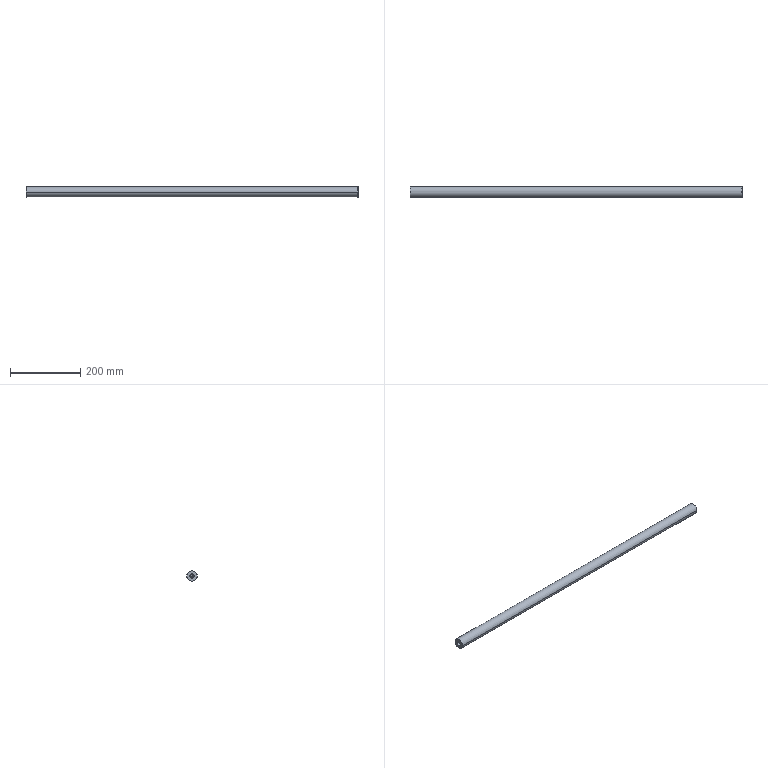Component | SolidWorks | FixedLengthRod-1 | 1 solid | 16 faces | box 944 x 30 x 30 mm | volume 659289 mm3 | cone 8 | cylinder 6 | plane 2 | commonest cylinder face diameters 12 x4 30 x2
build123d program:
from build123d import *

# Parameters (mm, degrees)
SKETCH1_R              = 15
BOSS_EXTRUDE1_DEPTH    = 944
CHAMFER1_SIZE          = 0.5
M14_TAPPED_HOLE1_D     = 12
M14_TAPPED_HOLE1_DEPTH = 34
M14_TAPPED_HOLE1_TIP   = 3.605
M14_TAPPED_HOLE2_D     = 12
M14_TAPPED_HOLE2_DEPTH = 34
M14_TAPPED_HOLE2_TIP   = 3.605


with BuildPart() as part:
    # Sketch1 → Boss-Extrude1 (new body)
    with BuildSketch(Plane.XY):
        Circle(SKETCH1_R)
    extrude(amount=BOSS_EXTRUDE1_DEPTH)

    # Chamfer1
    chamfer1_edges = [part.edges().sort_by_distance(p)[0] for p in [
        (-15, 0, 0),
        (-15, 0, 944),
    ]]
    chamfer(chamfer1_edges, length=CHAMFER1_SIZE)

    # M14 Tapped Hole1
    with Locations(Plane(origin=(0, 0, 0), x_dir=(-1, 0, 0), z_dir=(0, 0, -1))):
        with Locations((0, 0)):
            Hole(M14_TAPPED_HOLE1_D / 2, depth=M14_TAPPED_HOLE1_DEPTH)
            with Locations((0, 0, -(M14_TAPPED_HOLE1_DEPTH + M14_TAPPED_HOLE1_TIP / 2))):  # 118° drill point
                Cone(0, M14_TAPPED_HOLE1_D / 2, M14_TAPPED_HOLE1_TIP, mode=Mode.SUBTRACT)

    # M14 Tapped Hole2
    with Locations(Plane.XY.offset(944)):
        with Locations((0, 0)):
            Hole(M14_TAPPED_HOLE2_D / 2, depth=M14_TAPPED_HOLE2_DEPTH)
            with Locations((0, 0, -(M14_TAPPED_HOLE2_DEPTH + M14_TAPPED_HOLE2_TIP / 2))):  # 118° drill point
                Cone(0, M14_TAPPED_HOLE2_D / 2, M14_TAPPED_HOLE2_TIP, mode=Mode.SUBTRACT)


solid = part.part

# Placed as in the assembly
solid = solid.moved(Location((-625.02, -279.181, 155), (0, 90, 0)))
STEP:
#1=CARTESIAN_POINT('',(-23.269,-11.228,6.102));
#2=VERTEX_POINT('',#1);
#3=CARTESIAN_POINT('',(-23.269,-10.755,6.102));
#4=VERTEX_POINT('',#3);
#5=CARTESIAN_POINT('',(-23.269,-10.991,6.102));
#6=DIRECTION('',(-1.,0.,0.));
#7=DIRECTION('',(0.,1.,0.));
#8=AXIS2_PLACEMENT_3D('',#5,#6,#7);
#9=CIRCLE('',#8,0.2362);
#10=EDGE_CURVE('',#2,#4,#9,.T.);
#11=ORIENTED_EDGE('',*,*,#10,.F.);
#12=CARTESIAN_POINT('',(-24.607,-11.228,6.102));
#13=VERTEX_POINT('',#12);
#14=CARTESIAN_POINT('',(-24.607,-11.228,6.102));
#15=DIRECTION('',(-1.,0.,0.));
#16=VECTOR('',#15,39.37);
#17=LINE('',#14,#16);
#18=EDGE_CURVE('',#2,#13,#17,.T.);
#19=ORIENTED_EDGE('',*,*,#18,.T.);
#20=CARTESIAN_POINT('',(-24.607,-10.755,6.102));
#21=VERTEX_POINT('',#20);
#22=CARTESIAN_POINT('',(-24.607,-10.991,6.102));
#23=DIRECTION('',(-1.,0.,0.));
#24=DIRECTION('',(0.,1.,0.));
#25=AXIS2_PLACEMENT_3D('',#22,#23,#24);
#26=CIRCLE('',#25,0.2362);
#27=EDGE_CURVE('',#13,#21,#26,.T.);
#28=ORIENTED_EDGE('',*,*,#27,.T.);
#29=CARTESIAN_POINT('',(-24.607,-10.755,6.102));
#30=DIRECTION('',(-1.,0.,0.));
#31=VECTOR('',#30,39.37);
#32=LINE('',#29,#31);
#33=EDGE_CURVE('',#4,#21,#32,.T.);
#34=ORIENTED_EDGE('',*,*,#33,.F.);
#35=EDGE_LOOP('',(#11,#19,#28,#34));
#36=FACE_OUTER_BOUND('',#35,.T.);
#37=CARTESIAN_POINT('',(-24.607,-10.991,6.102));
#38=DIRECTION('',(-1.,0.,0.));
#39=DIRECTION('',(0.,1.,0.));
#40=AXIS2_PLACEMENT_3D('',#37,#38,#39);
#41=CYLINDRICAL_SURFACE('',#40,0.2362);
#42=ADVANCED_FACE('',(#36),#41,.F.);
#43=CARTESIAN_POINT('',(-23.127,-10.991,6.102));
#44=VERTEX_POINT('',#43);
#45=CARTESIAN_POINT('',(-23.269,-10.755,6.102));
#46=DIRECTION('',(-0.515,0.8572,0.));
#47=VECTOR('',#46,39.37);
#48=LINE('',#45,#47);
#49=EDGE_CURVE('',#44,#4,#48,.T.);
#50=ORIENTED_EDGE('',*,*,#49,.F.);
#51=CARTESIAN_POINT('',(-23.269,-11.228,6.102));
#52=DIRECTION('',(-0.515,-0.8572,-0.));
#53=VECTOR('',#52,39.37);
#54=LINE('',#51,#53);
#55=EDGE_CURVE('',#44,#2,#54,.T.);
#56=ORIENTED_EDGE('',*,*,#55,.T.);
#57=ORIENTED_EDGE('',*,*,#10,.T.);
#58=EDGE_LOOP('',(#50,#56,#57));
#59=FACE_OUTER_BOUND('',#58,.T.);
#60=CARTESIAN_POINT('',(-23.269,-10.991,6.102));
#61=DIRECTION('',(-1.,0.,0.));
#62=DIRECTION('',(0.,1.,0.));
#63=AXIS2_PLACEMENT_3D('',#60,#61,#62);
#64=CONICAL_SURFACE('',#63,0.2362,1.03);
#65=ADVANCED_FACE('',(#59),#64,.F.);
#66=CARTESIAN_POINT('',(11.22,-10.755,6.102));
#67=VERTEX_POINT('',#66);
#68=CARTESIAN_POINT('',(11.22,-11.228,6.102));
#69=VERTEX_POINT('',#68);
#70=CARTESIAN_POINT('',(11.22,-10.991,6.102));
#71=DIRECTION('',(1.,0.,0.));
#72=DIRECTION('',(0.,-1.,0.));
#73=AXIS2_PLACEMENT_3D('',#70,#71,#72);
#74=CIRCLE('',#73,0.2362);
#75=EDGE_CURVE('',#67,#69,#74,.T.);
#76=ORIENTED_EDGE('',*,*,#75,.F.);
#77=CARTESIAN_POINT('',(12.558,-10.755,6.102));
#78=VERTEX_POINT('',#77);
#79=CARTESIAN_POINT('',(12.558,-10.755,6.102));
#80=DIRECTION('',(1.,0.,0.));
#81=VECTOR('',#80,39.37);
#82=LINE('',#79,#81);
#83=EDGE_CURVE('',#67,#78,#82,.T.);
#84=ORIENTED_EDGE('',*,*,#83,.T.);
#85=CARTESIAN_POINT('',(12.558,-11.228,6.102));
#86=VERTEX_POINT('',#85);
#87=CARTESIAN_POINT('',(12.558,-10.991,6.102));
#88=DIRECTION('',(1.,0.,0.));
#89=DIRECTION('',(0.,-1.,0.));
#90=AXIS2_PLACEMENT_3D('',#87,#88,#89);
#91=CIRCLE('',#90,0.2362);
#92=EDGE_CURVE('',#78,#86,#91,.T.);
#93=ORIENTED_EDGE('',*,*,#92,.T.);
#94=CARTESIAN_POINT('',(12.558,-11.228,6.102));
#95=DIRECTION('',(1.,0.,0.));
#96=VECTOR('',#95,39.37);
#97=LINE('',#94,#96);
#98=EDGE_CURVE('',#69,#86,#97,.T.);
#99=ORIENTED_EDGE('',*,*,#98,.F.);
#100=EDGE_LOOP('',(#76,#84,#93,#99));
#101=FACE_OUTER_BOUND('',#100,.T.);
#102=CARTESIAN_POINT('',(12.558,-10.991,6.102));
#103=DIRECTION('',(1.,0.,0.));
#104=DIRECTION('',(0.,-1.,0.));
#105=AXIS2_PLACEMENT_3D('',#102,#103,#104);
#106=CYLINDRICAL_SURFACE('',#105,0.2362);
#107=ADVANCED_FACE('',(#101),#106,.F.);
#108=CARTESIAN_POINT('',(11.078,-10.991,6.102));
#109=VERTEX_POINT('',#108);
#110=CARTESIAN_POINT('',(11.22,-11.228,6.102));
#111=DIRECTION('',(0.515,-0.8572,-0.));
#112=VECTOR('',#111,39.37);
#113=LINE('',#110,#112);
#114=EDGE_CURVE('',#109,#69,#113,.T.);
#115=ORIENTED_EDGE('',*,*,#114,.F.);
#116=CARTESIAN_POINT('',(11.22,-10.755,6.102));
#117=DIRECTION('',(0.515,0.8572,0.));
#118=VECTOR('',#117,39.37);
#119=LINE('',#116,#118);
#120=EDGE_CURVE('',#109,#67,#119,.T.);
#121=ORIENTED_EDGE('',*,*,#120,.T.);
#122=ORIENTED_EDGE('',*,*,#75,.T.);
#123=EDGE_LOOP('',(#115,#121,#122));
#124=FACE_OUTER_BOUND('',#123,.T.);
#125=CARTESIAN_POINT('',(11.22,-10.991,6.102));
#126=DIRECTION('',(1.,0.,0.));
#127=DIRECTION('',(0.,-1.,0.));
#128=AXIS2_PLACEMENT_3D('',#125,#126,#127);
#129=CONICAL_SURFACE('',#128,0.2362,1.03);
#130=ADVANCED_FACE('',(#124),#129,.F.);
#131=CARTESIAN_POINT('',(-24.607,-10.421,6.102));
#132=VERTEX_POINT('',#131);
#133=CARTESIAN_POINT('',(-24.607,-11.562,6.102));
#134=VERTEX_POINT('',#133);
#135=CARTESIAN_POINT('',(-24.607,-10.991,6.102));
#136=DIRECTION('',(-1.,0.,0.));
#137=DIRECTION('',(0.,1.,0.));
#138=AXIS2_PLACEMENT_3D('',#135,#136,#137);
#139=CIRCLE('',#138,0.5709);
#140=EDGE_CURVE('',#132,#134,#139,.T.);
#141=ORIENTED_EDGE('',*,*,#140,.F.);
#142=CARTESIAN_POINT('',(-24.587,-10.401,6.102));
#143=VERTEX_POINT('',#142);
#144=CARTESIAN_POINT('',(-24.607,-10.421,6.102));
#145=DIRECTION('',(0.7071,0.7071,0.));
#146=VECTOR('',#145,39.37);
#147=LINE('',#144,#146);
#148=EDGE_CURVE('',#132,#143,#147,.T.);
#149=ORIENTED_EDGE('',*,*,#148,.T.);
#150=CARTESIAN_POINT('',(-24.587,-11.582,6.102));
#151=VERTEX_POINT('',#150);
#152=CARTESIAN_POINT('',(-24.587,-10.991,6.102));
#153=DIRECTION('',(1.,0.,0.));
#154=DIRECTION('',(0.,1.,0.));
#155=AXIS2_PLACEMENT_3D('',#152,#153,#154);
#156=CIRCLE('',#155,0.5906);
#157=EDGE_CURVE('',#151,#143,#156,.T.);
#158=ORIENTED_EDGE('',*,*,#157,.F.);
#159=CARTESIAN_POINT('',(-24.607,-11.562,6.102));
#160=DIRECTION('',(0.7071,-0.7071,-0.));
#161=VECTOR('',#160,39.37);
#162=LINE('',#159,#161);
#163=EDGE_CURVE('',#134,#151,#162,.T.);
#164=ORIENTED_EDGE('',*,*,#163,.F.);
#165=EDGE_LOOP('',(#141,#149,#158,#164));
#166=FACE_OUTER_BOUND('',#165,.T.);
#167=CARTESIAN_POINT('',(-24.607,-10.991,6.102));
#168=DIRECTION('',(1.,0.,0.));
#169=DIRECTION('',(0.,-1.,-0.));
#170=AXIS2_PLACEMENT_3D('',#167,#168,#169);
#171=CONICAL_SURFACE('',#170,0.5709,0.7854);
#172=ADVANCED_FACE('',(#166),#171,.T.);
#173=CARTESIAN_POINT('',(12.558,-11.562,6.102));
#174=VERTEX_POINT('',#173);
#175=CARTESIAN_POINT('',(12.558,-10.421,6.102));
#176=VERTEX_POINT('',#175);
#177=CARTESIAN_POINT('',(12.558,-10.991,6.102));
#178=DIRECTION('',(1.,0.,0.));
#179=DIRECTION('',(0.,1.,0.));
#180=AXIS2_PLACEMENT_3D('',#177,#178,#179);
#181=CIRCLE('',#180,0.5709);
#182=EDGE_CURVE('',#174,#176,#181,.T.);
#183=ORIENTED_EDGE('',*,*,#182,.F.);
#184=CARTESIAN_POINT('',(12.539,-11.582,6.102));
#185=VERTEX_POINT('',#184);
#186=CARTESIAN_POINT('',(12.539,-11.582,6.102));
#187=DIRECTION('',(-0.7071,-0.7071,-0.));
#188=VECTOR('',#187,39.37);
#189=LINE('',#186,#188);
#190=EDGE_CURVE('',#174,#185,#189,.T.);
#191=ORIENTED_EDGE('',*,*,#190,.T.);
#192=CARTESIAN_POINT('',(12.539,-10.401,6.102));
#193=VERTEX_POINT('',#192);
#194=CARTESIAN_POINT('',(12.539,-10.991,6.102));
#195=DIRECTION('',(-1.,0.,0.));
#196=DIRECTION('',(0.,1.,0.));
#197=AXIS2_PLACEMENT_3D('',#194,#195,#196);
#198=CIRCLE('',#197,0.5906);
#199=EDGE_CURVE('',#193,#185,#198,.T.);
#200=ORIENTED_EDGE('',*,*,#199,.F.);
#201=CARTESIAN_POINT('',(12.539,-10.401,6.102));
#202=DIRECTION('',(-0.7071,0.7071,0.));
#203=VECTOR('',#202,39.37);
#204=LINE('',#201,#203);
#205=EDGE_CURVE('',#176,#193,#204,.T.);
#206=ORIENTED_EDGE('',*,*,#205,.F.);
#207=EDGE_LOOP('',(#183,#191,#200,#206));
#208=FACE_OUTER_BOUND('',#207,.T.);
#209=CARTESIAN_POINT('',(12.539,-10.991,6.102));
#210=DIRECTION('',(-1.,0.,0.));
#211=DIRECTION('',(0.,1.,0.));
#212=AXIS2_PLACEMENT_3D('',#209,#210,#211);
#213=CONICAL_SURFACE('',#212,0.5906,0.7854);
#214=ADVANCED_FACE('',(#208),#213,.T.);
#215=ORIENTED_EDGE('',*,*,#157,.T.);
#216=CARTESIAN_POINT('',(-24.607,-10.401,6.102));
#217=DIRECTION('',(1.,0.,0.));
#218=VECTOR('',#217,39.37);
#219=LINE('',#216,#218);
#220=EDGE_CURVE('',#143,#193,#219,.T.);
#221=ORIENTED_EDGE('',*,*,#220,.T.);
#222=ORIENTED_EDGE('',*,*,#199,.T.);
#223=CARTESIAN_POINT('',(-24.607,-11.582,6.102));
#224=DIRECTION('',(1.,0.,0.));
#225=VECTOR('',#224,39.37);
#226=LINE('',#223,#225);
#227=EDGE_CURVE('',#151,#185,#226,.T.);
#228=ORIENTED_EDGE('',*,*,#227,.F.);
#229=EDGE_LOOP('',(#215,#221,#222,#228));
#230=FACE_OUTER_BOUND('',#229,.T.);
#231=CARTESIAN_POINT('',(-24.607,-10.991,6.102));
#232=DIRECTION('',(1.,0.,0.));
#233=DIRECTION('',(0.,-1.,-0.));
#234=AXIS2_PLACEMENT_3D('',#231,#232,#233);
#235=CYLINDRICAL_SURFACE('',#234,0.5906);
#236=ADVANCED_FACE('',(#230),#235,.T.);
#237=ORIENTED_EDGE('',*,*,#220,.F.);
#238=CARTESIAN_POINT('',(-24.587,-10.991,6.102));
#239=DIRECTION('',(1.,0.,0.));
#240=DIRECTION('',(0.,1.,0.));
#241=AXIS2_PLACEMENT_3D('',#238,#239,#240);
#242=CIRCLE('',#241,0.5906);
#243=EDGE_CURVE('',#143,#151,#242,.T.);
#244=ORIENTED_EDGE('',*,*,#243,.T.);
#245=ORIENTED_EDGE('',*,*,#227,.T.);
#246=CARTESIAN_POINT('',(12.539,-10.991,6.102));
#247=DIRECTION('',(-1.,0.,0.));
#248=DIRECTION('',(0.,1.,0.));
#249=AXIS2_PLACEMENT_3D('',#246,#247,#248);
#250=CIRCLE('',#249,0.5906);
#251=EDGE_CURVE('',#185,#193,#250,.T.);
#252=ORIENTED_EDGE('',*,*,#251,.T.);
#253=EDGE_LOOP('',(#237,#244,#245,#252));
#254=FACE_OUTER_BOUND('',#253,.T.);
#255=CARTESIAN_POINT('',(-24.607,-10.991,6.102));
#256=DIRECTION('',(1.,0.,0.));
#257=DIRECTION('',(0.,-1.,-0.));
#258=AXIS2_PLACEMENT_3D('',#255,#256,#257);
#259=CYLINDRICAL_SURFACE('',#258,0.5906);
#260=ADVANCED_FACE('',(#254),#259,.T.);
#261=CARTESIAN_POINT('',(-24.607,-10.991,6.102));
#262=DIRECTION('',(-1.,0.,0.));
#263=DIRECTION('',(0.,1.,0.));
#264=AXIS2_PLACEMENT_3D('',#261,#262,#263);
#265=CIRCLE('',#264,0.2362);
#266=EDGE_CURVE('',#21,#13,#265,.T.);
#267=ORIENTED_EDGE('',*,*,#266,.F.);
#268=ORIENTED_EDGE('',*,*,#27,.F.);
#269=EDGE_LOOP('',(#267,#268));
#270=FACE_BOUND('',#269,.T.);
#271=CARTESIAN_POINT('',(-24.607,-10.991,6.102));
#272=DIRECTION('',(-1.,0.,0.));
#273=DIRECTION('',(0.,1.,0.));
#274=AXIS2_PLACEMENT_3D('',#271,#272,#273);
#275=CIRCLE('',#274,0.5709);
#276=EDGE_CURVE('',#134,#132,#275,.T.);
#277=ORIENTED_EDGE('',*,*,#276,.T.);
#278=ORIENTED_EDGE('',*,*,#140,.T.);
#279=EDGE_LOOP('',(#277,#278));
#280=FACE_OUTER_BOUND('',#279,.T.);
#281=CARTESIAN_POINT('',(-24.607,-10.991,6.102));
#282=DIRECTION('',(-1.,0.,0.));
#283=DIRECTION('',(0.,1.,0.));
#284=AXIS2_PLACEMENT_3D('',#281,#282,#283);
#285=PLANE('',#284);
#286=ADVANCED_FACE('',(#270,#280),#285,.T.);
#287=CARTESIAN_POINT('',(12.558,-10.991,6.102));
#288=DIRECTION('',(1.,0.,0.));
#289=DIRECTION('',(0.,-1.,0.));
#290=AXIS2_PLACEMENT_3D('',#287,#288,#289);
#291=CIRCLE('',#290,0.2362);
#292=EDGE_CURVE('',#86,#78,#291,.T.);
#293=ORIENTED_EDGE('',*,*,#292,.F.);
#294=ORIENTED_EDGE('',*,*,#92,.F.);
#295=EDGE_LOOP('',(#293,#294));
#296=FACE_BOUND('',#295,.T.);
#297=CARTESIAN_POINT('',(12.558,-10.991,6.102));
#298=DIRECTION('',(1.,0.,0.));
#299=DIRECTION('',(0.,1.,0.));
#300=AXIS2_PLACEMENT_3D('',#297,#298,#299);
#301=CIRCLE('',#300,0.5709);
#302=EDGE_CURVE('',#176,#174,#301,.T.);
#303=ORIENTED_EDGE('',*,*,#302,.T.);
#304=ORIENTED_EDGE('',*,*,#182,.T.);
#305=EDGE_LOOP('',(#303,#304));
#306=FACE_OUTER_BOUND('',#305,.T.);
#307=CARTESIAN_POINT('',(12.558,-10.991,6.102));
#308=DIRECTION('',(-1.,0.,0.));
#309=DIRECTION('',(0.,1.,0.));
#310=AXIS2_PLACEMENT_3D('',#307,#308,#309);
#311=PLANE('',#310);
#312=ADVANCED_FACE('',(#296,#306),#311,.F.);
#313=ORIENTED_EDGE('',*,*,#190,.F.);
#314=ORIENTED_EDGE('',*,*,#302,.F.);
#315=ORIENTED_EDGE('',*,*,#205,.T.);
#316=ORIENTED_EDGE('',*,*,#251,.F.);
#317=EDGE_LOOP('',(#313,#314,#315,#316));
#318=FACE_OUTER_BOUND('',#317,.T.);
#319=CARTESIAN_POINT('',(12.539,-10.991,6.102));
#320=DIRECTION('',(-1.,0.,0.));
#321=DIRECTION('',(0.,1.,0.));
#322=AXIS2_PLACEMENT_3D('',#319,#320,#321);
#323=CONICAL_SURFACE('',#322,0.5906,0.7854);
#324=ADVANCED_FACE('',(#318),#323,.T.);
#325=ORIENTED_EDGE('',*,*,#148,.F.);
#326=ORIENTED_EDGE('',*,*,#276,.F.);
#327=ORIENTED_EDGE('',*,*,#163,.T.);
#328=ORIENTED_EDGE('',*,*,#243,.F.);
#329=EDGE_LOOP('',(#325,#326,#327,#328));
#330=FACE_OUTER_BOUND('',#329,.T.);
#331=CARTESIAN_POINT('',(-24.607,-10.991,6.102));
#332=DIRECTION('',(1.,0.,0.));
#333=DIRECTION('',(0.,-1.,-0.));
#334=AXIS2_PLACEMENT_3D('',#331,#332,#333);
#335=CONICAL_SURFACE('',#334,0.5709,0.7854);
#336=ADVANCED_FACE('',(#330),#335,.T.);
#337=ORIENTED_EDGE('',*,*,#120,.F.);
#338=ORIENTED_EDGE('',*,*,#114,.T.);
#339=CARTESIAN_POINT('',(11.22,-10.991,6.102));
#340=DIRECTION('',(1.,0.,0.));
#341=DIRECTION('',(0.,-1.,0.));
#342=AXIS2_PLACEMENT_3D('',#339,#340,#341);
#343=CIRCLE('',#342,0.2362);
#344=EDGE_CURVE('',#69,#67,#343,.T.);
#345=ORIENTED_EDGE('',*,*,#344,.T.);
#346=EDGE_LOOP('',(#337,#338,#345));
#347=FACE_OUTER_BOUND('',#346,.T.);
#348=CARTESIAN_POINT('',(11.22,-10.991,6.102));
#349=DIRECTION('',(1.,0.,0.));
#350=DIRECTION('',(0.,-1.,0.));
#351=AXIS2_PLACEMENT_3D('',#348,#349,#350);
#352=CONICAL_SURFACE('',#351,0.2362,1.03);
#353=ADVANCED_FACE('',(#347),#352,.F.);
#354=ORIENTED_EDGE('',*,*,#83,.F.);
#355=ORIENTED_EDGE('',*,*,#344,.F.);
#356=ORIENTED_EDGE('',*,*,#98,.T.);
#357=ORIENTED_EDGE('',*,*,#292,.T.);
#358=EDGE_LOOP('',(#354,#355,#356,#357));
#359=FACE_OUTER_BOUND('',#358,.T.);
#360=CARTESIAN_POINT('',(12.558,-10.991,6.102));
#361=DIRECTION('',(1.,0.,0.));
#362=DIRECTION('',(0.,-1.,0.));
#363=AXIS2_PLACEMENT_3D('',#360,#361,#362);
#364=CYLINDRICAL_SURFACE('',#363,0.2362);
#365=ADVANCED_FACE('',(#359),#364,.F.);
#366=ORIENTED_EDGE('',*,*,#55,.F.);
#367=ORIENTED_EDGE('',*,*,#49,.T.);
#368=CARTESIAN_POINT('',(-23.269,-10.991,6.102));
#369=DIRECTION('',(-1.,0.,0.));
#370=DIRECTION('',(0.,1.,0.));
#371=AXIS2_PLACEMENT_3D('',#368,#369,#370);
#372=CIRCLE('',#371,0.2362);
#373=EDGE_CURVE('',#4,#2,#372,.T.);
#374=ORIENTED_EDGE('',*,*,#373,.T.);
#375=EDGE_LOOP('',(#366,#367,#374));
#376=FACE_OUTER_BOUND('',#375,.T.);
#377=CARTESIAN_POINT('',(-23.269,-10.991,6.102));
#378=DIRECTION('',(-1.,0.,0.));
#379=DIRECTION('',(0.,1.,0.));
#380=AXIS2_PLACEMENT_3D('',#377,#378,#379);
#381=CONICAL_SURFACE('',#380,0.2362,1.03);
#382=ADVANCED_FACE('',(#376),#381,.F.);
#383=ORIENTED_EDGE('',*,*,#18,.F.);
#384=ORIENTED_EDGE('',*,*,#373,.F.);
#385=ORIENTED_EDGE('',*,*,#33,.T.);
#386=ORIENTED_EDGE('',*,*,#266,.T.);
#387=EDGE_LOOP('',(#383,#384,#385,#386));
#388=FACE_OUTER_BOUND('',#387,.T.);
#389=CARTESIAN_POINT('',(-24.607,-10.991,6.102));
#390=DIRECTION('',(-1.,0.,0.));
#391=DIRECTION('',(0.,1.,0.));
#392=AXIS2_PLACEMENT_3D('',#389,#390,#391);
#393=CYLINDRICAL_SURFACE('',#392,0.2362);
#394=ADVANCED_FACE('',(#388),#393,.F.);
#395=CLOSED_SHELL('',(#42,#65,#107,#130,#172,#214,#236,#260,#286,#312,#324,#336,#353,#365,#382,#394));
#396=MANIFOLD_SOLID_BREP('',#395);
#397=CARTESIAN_POINT('',(0.,0.,0.));
#398=DIRECTION('',(0.,0.,1.));
#399=DIRECTION('',(1.,0.,0.));
#400=AXIS2_PLACEMENT_3D('',#397,#398,#399);
#401=(LENGTH_UNIT()NAMED_UNIT(*)SI_UNIT($,.METRE.));
#402=LENGTH_MEASURE_WITH_UNIT(LENGTH_MEASURE(0.0254),#401);
#403=DIMENSIONAL_EXPONENTS(1.,0.,0.,0.,0.,0.,0.);
#404=(CONVERSION_BASED_UNIT('',#402)LENGTH_UNIT()NAMED_UNIT(#403));
#405=UNCERTAINTY_MEASURE_WITH_UNIT(LENGTH_MEASURE(0.00001),#404,'','');
#406=(NAMED_UNIT(*)PLANE_ANGLE_UNIT()SI_UNIT($,.RADIAN.));
#407=(NAMED_UNIT(*)SI_UNIT($,.STERADIAN.)SOLID_ANGLE_UNIT());
#408=(GEOMETRIC_REPRESENTATION_CONTEXT(3)GLOBAL_UNCERTAINTY_ASSIGNED_CONTEXT((#405))GLOBAL_UNIT_ASSIGNED_CONTEXT((#404,#406,#407))REPRESENTATION_CONTEXT('',''));
#409=ADVANCED_BREP_SHAPE_REPRESENTATION('',(#396,#400),#408);
#410=COLOUR_RGB('',0.7922,0.8196,0.9333);
#411=FILL_AREA_STYLE_COLOUR('',#410);
#412=FILL_AREA_STYLE('',(#411));
#413=SURFACE_STYLE_FILL_AREA(#412);
#414=SURFACE_SIDE_STYLE('',(#413));
#415=SURFACE_STYLE_USAGE(.BOTH.,#414);
#416=PRESENTATION_STYLE_ASSIGNMENT((#415));
#417=STYLED_ITEM('',(#416),#396);
#418=PRESENTATION_LAYER_ASSIGNMENT('','',(#417));
#419=(LENGTH_UNIT()NAMED_UNIT(*)SI_UNIT($,.METRE.));
#420=LENGTH_MEASURE_WITH_UNIT(LENGTH_MEASURE(0.0254),#419);
#421=DIMENSIONAL_EXPONENTS(1.,0.,0.,0.,0.,0.,0.);
#422=(CONVERSION_BASED_UNIT('',#420)LENGTH_UNIT()NAMED_UNIT(#421));
#423=UNCERTAINTY_MEASURE_WITH_UNIT(LENGTH_MEASURE(0.00001),#422,'','');
#424=(NAMED_UNIT(*)PLANE_ANGLE_UNIT()SI_UNIT($,.RADIAN.));
#425=(NAMED_UNIT(*)SI_UNIT($,.STERADIAN.)SOLID_ANGLE_UNIT());
#426=(GEOMETRIC_REPRESENTATION_CONTEXT(3)GLOBAL_UNCERTAINTY_ASSIGNED_CONTEXT((#423))GLOBAL_UNIT_ASSIGNED_CONTEXT((#422,#424,#425))REPRESENTATION_CONTEXT('',''));
#427=MECHANICAL_DESIGN_GEOMETRIC_PRESENTATION_REPRESENTATION('',(#417),#426);